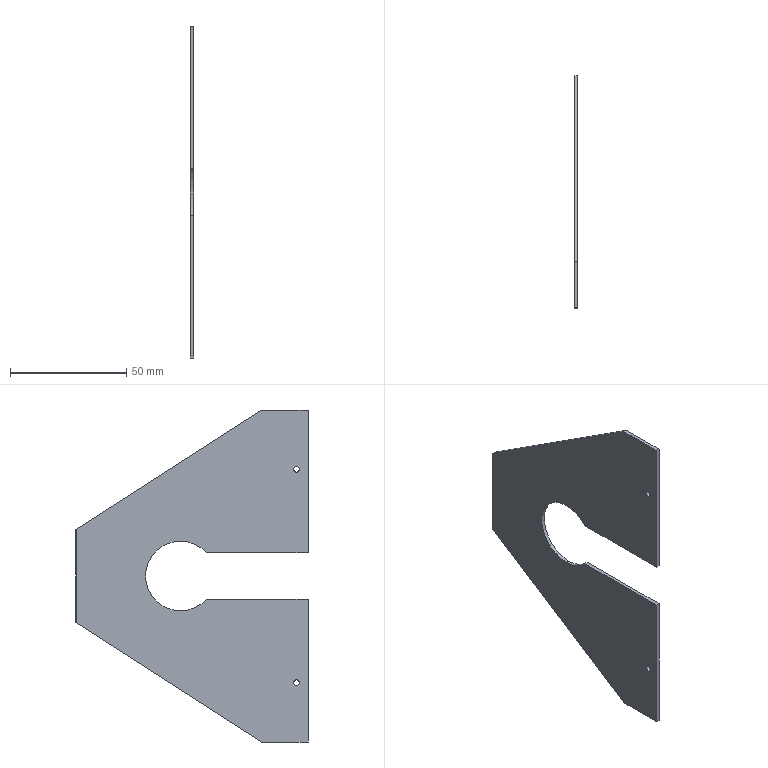Component | SolidWorks | Lampshade-1_Lampshade1-2 | 1 solid | 20 faces | box 1.5 x 100 x 143 mm | volume 12957 mm3 | plane 13 | cylinder 7 | commonest cylinder face diameters 2.5 x4 30 x3
STEP:
#1=CARTESIAN_POINT('',(-6.136,-3.389,1.388));
#2=VERTEX_POINT('',#1);
#3=CARTESIAN_POINT('',(-6.136,-3.389,1.289));
#4=VERTEX_POINT('',#3);
#5=CARTESIAN_POINT('',(-6.136,-3.389,1.339));
#6=DIRECTION('',(1.,-0.,0.));
#7=DIRECTION('',(0.,0.,-1.));
#8=AXIS2_PLACEMENT_3D('',#5,#6,#7);
#9=CIRCLE('',#8,0.04921);
#10=EDGE_CURVE('',#2,#4,#9,.T.);
#11=ORIENTED_EDGE('',*,*,#10,.F.);
#12=CARTESIAN_POINT('',(-6.077,-3.389,1.388));
#13=VERTEX_POINT('',#12);
#14=CARTESIAN_POINT('',(-6.136,-3.389,1.388));
#15=DIRECTION('',(1.,-0.,0.));
#16=VECTOR('',#15,39.37);
#17=LINE('',#14,#16);
#18=EDGE_CURVE('',#2,#13,#17,.T.);
#19=ORIENTED_EDGE('',*,*,#18,.T.);
#20=CARTESIAN_POINT('',(-6.077,-3.389,1.289));
#21=VERTEX_POINT('',#20);
#22=CARTESIAN_POINT('',(-6.077,-3.389,1.339));
#23=DIRECTION('',(1.,-0.,0.));
#24=DIRECTION('',(0.,0.,-1.));
#25=AXIS2_PLACEMENT_3D('',#22,#23,#24);
#26=CIRCLE('',#25,0.04921);
#27=EDGE_CURVE('',#13,#21,#26,.T.);
#28=ORIENTED_EDGE('',*,*,#27,.T.);
#29=CARTESIAN_POINT('',(-6.136,-3.389,1.289));
#30=DIRECTION('',(1.,-0.,0.));
#31=VECTOR('',#30,39.37);
#32=LINE('',#29,#31);
#33=EDGE_CURVE('',#4,#21,#32,.T.);
#34=ORIENTED_EDGE('',*,*,#33,.F.);
#35=EDGE_LOOP('',(#11,#19,#28,#34));
#36=FACE_OUTER_BOUND('',#35,.T.);
#37=CARTESIAN_POINT('',(-6.136,-3.389,1.339));
#38=DIRECTION('',(1.,-0.,0.));
#39=DIRECTION('',(0.,0.,-1.));
#40=AXIS2_PLACEMENT_3D('',#37,#38,#39);
#41=CYLINDRICAL_SURFACE('',#40,0.04921);
#42=ADVANCED_FACE('',(#36),#41,.F.);
#43=CARTESIAN_POINT('',(-6.136,-3.389,5.01));
#44=VERTEX_POINT('',#43);
#45=CARTESIAN_POINT('',(-6.136,-3.389,4.911));
#46=VERTEX_POINT('',#45);
#47=CARTESIAN_POINT('',(-6.136,-3.389,4.961));
#48=DIRECTION('',(1.,-0.,0.));
#49=DIRECTION('',(0.,0.,-1.));
#50=AXIS2_PLACEMENT_3D('',#47,#48,#49);
#51=CIRCLE('',#50,0.04921);
#52=EDGE_CURVE('',#44,#46,#51,.T.);
#53=ORIENTED_EDGE('',*,*,#52,.F.);
#54=CARTESIAN_POINT('',(-6.077,-3.389,5.01));
#55=VERTEX_POINT('',#54);
#56=CARTESIAN_POINT('',(-6.136,-3.389,5.01));
#57=DIRECTION('',(1.,-0.,0.));
#58=VECTOR('',#57,39.37);
#59=LINE('',#56,#58);
#60=EDGE_CURVE('',#44,#55,#59,.T.);
#61=ORIENTED_EDGE('',*,*,#60,.T.);
#62=CARTESIAN_POINT('',(-6.077,-3.389,4.911));
#63=VERTEX_POINT('',#62);
#64=CARTESIAN_POINT('',(-6.077,-3.389,4.961));
#65=DIRECTION('',(1.,-0.,0.));
#66=DIRECTION('',(0.,0.,-1.));
#67=AXIS2_PLACEMENT_3D('',#64,#65,#66);
#68=CIRCLE('',#67,0.04921);
#69=EDGE_CURVE('',#55,#63,#68,.T.);
#70=ORIENTED_EDGE('',*,*,#69,.T.);
#71=CARTESIAN_POINT('',(-6.136,-3.389,4.911));
#72=DIRECTION('',(1.,-0.,0.));
#73=VECTOR('',#72,39.37);
#74=LINE('',#71,#73);
#75=EDGE_CURVE('',#46,#63,#74,.T.);
#76=ORIENTED_EDGE('',*,*,#75,.F.);
#77=EDGE_LOOP('',(#53,#61,#70,#76));
#78=FACE_OUTER_BOUND('',#77,.T.);
#79=CARTESIAN_POINT('',(-6.136,-3.389,4.961));
#80=DIRECTION('',(1.,-0.,0.));
#81=DIRECTION('',(0.,0.,-1.));
#82=AXIS2_PLACEMENT_3D('',#79,#80,#81);
#83=CYLINDRICAL_SURFACE('',#82,0.04921);
#84=ADVANCED_FACE('',(#78),#83,.F.);
#85=CARTESIAN_POINT('',(-6.136,-1.861,3.543));
#86=VERTEX_POINT('',#85);
#87=CARTESIAN_POINT('',(-6.136,-1.421,3.74));
#88=VERTEX_POINT('',#87);
#89=CARTESIAN_POINT('',(-6.136,-1.421,3.15));
#90=DIRECTION('',(-1.,0.,0.));
#91=DIRECTION('',(0.,0.,-1.));
#92=AXIS2_PLACEMENT_3D('',#89,#90,#91);
#93=CIRCLE('',#92,0.5906);
#94=EDGE_CURVE('',#86,#88,#93,.T.);
#95=ORIENTED_EDGE('',*,*,#94,.T.);
#96=CARTESIAN_POINT('',(-6.077,-1.421,3.74));
#97=VERTEX_POINT('',#96);
#98=CARTESIAN_POINT('',(-6.136,-1.421,3.74));
#99=DIRECTION('',(1.,-0.,0.));
#100=VECTOR('',#99,39.37);
#101=LINE('',#98,#100);
#102=EDGE_CURVE('',#88,#97,#101,.T.);
#103=ORIENTED_EDGE('',*,*,#102,.T.);
#104=CARTESIAN_POINT('',(-6.077,-1.861,3.543));
#105=VERTEX_POINT('',#104);
#106=CARTESIAN_POINT('',(-6.077,-1.421,3.15));
#107=DIRECTION('',(-1.,0.,0.));
#108=DIRECTION('',(0.,0.,-1.));
#109=AXIS2_PLACEMENT_3D('',#106,#107,#108);
#110=CIRCLE('',#109,0.5906);
#111=EDGE_CURVE('',#105,#97,#110,.T.);
#112=ORIENTED_EDGE('',*,*,#111,.F.);
#113=CARTESIAN_POINT('',(-6.136,-1.861,3.543));
#114=DIRECTION('',(1.,-0.,0.));
#115=VECTOR('',#114,39.37);
#116=LINE('',#113,#115);
#117=EDGE_CURVE('',#86,#105,#116,.T.);
#118=ORIENTED_EDGE('',*,*,#117,.F.);
#119=EDGE_LOOP('',(#95,#103,#112,#118));
#120=FACE_OUTER_BOUND('',#119,.T.);
#121=CARTESIAN_POINT('',(-6.136,-1.421,3.15));
#122=DIRECTION('',(1.,-0.,0.));
#123=DIRECTION('',(0.,0.,-1.));
#124=AXIS2_PLACEMENT_3D('',#121,#122,#123);
#125=CYLINDRICAL_SURFACE('',#124,0.5906);
#126=ADVANCED_FACE('',(#120),#125,.F.);
#127=ORIENTED_EDGE('',*,*,#102,.F.);
#128=CARTESIAN_POINT('',(-6.136,-1.421,2.559));
#129=VERTEX_POINT('',#128);
#130=CARTESIAN_POINT('',(-6.136,-1.421,3.15));
#131=DIRECTION('',(-1.,0.,0.));
#132=DIRECTION('',(0.,0.,-1.));
#133=AXIS2_PLACEMENT_3D('',#130,#131,#132);
#134=CIRCLE('',#133,0.5906);
#135=EDGE_CURVE('',#88,#129,#134,.T.);
#136=ORIENTED_EDGE('',*,*,#135,.T.);
#137=CARTESIAN_POINT('',(-6.077,-1.421,2.559));
#138=VERTEX_POINT('',#137);
#139=CARTESIAN_POINT('',(-6.136,-1.421,2.559));
#140=DIRECTION('',(1.,-0.,0.));
#141=VECTOR('',#140,39.37);
#142=LINE('',#139,#141);
#143=EDGE_CURVE('',#129,#138,#142,.T.);
#144=ORIENTED_EDGE('',*,*,#143,.T.);
#145=CARTESIAN_POINT('',(-6.077,-1.421,3.15));
#146=DIRECTION('',(-1.,0.,0.));
#147=DIRECTION('',(0.,0.,-1.));
#148=AXIS2_PLACEMENT_3D('',#145,#146,#147);
#149=CIRCLE('',#148,0.5906);
#150=EDGE_CURVE('',#97,#138,#149,.T.);
#151=ORIENTED_EDGE('',*,*,#150,.F.);
#152=EDGE_LOOP('',(#127,#136,#144,#151));
#153=FACE_OUTER_BOUND('',#152,.T.);
#154=CARTESIAN_POINT('',(-6.136,-1.421,3.15));
#155=DIRECTION('',(1.,-0.,0.));
#156=DIRECTION('',(0.,0.,-1.));
#157=AXIS2_PLACEMENT_3D('',#154,#155,#156);
#158=CYLINDRICAL_SURFACE('',#157,0.5906);
#159=ADVANCED_FACE('',(#153),#158,.F.);
#160=CARTESIAN_POINT('',(-6.128,0.3509,2.362));
#161=VERTEX_POINT('',#160);
#162=CARTESIAN_POINT('',(-6.085,0.3509,2.362));
#163=VERTEX_POINT('',#162);
#164=CARTESIAN_POINT('',(-6.136,0.3509,2.362));
#165=DIRECTION('',(1.,-0.,0.));
#166=VECTOR('',#165,39.37);
#167=LINE('',#164,#166);
#168=EDGE_CURVE('',#161,#163,#167,.T.);
#169=ORIENTED_EDGE('',*,*,#168,.T.);
#170=CARTESIAN_POINT('',(-6.077,0.343,2.357));
#171=VERTEX_POINT('',#170);
#172=CARTESIAN_POINT('',(-4.261,-1.473,1.188));
#173=DIRECTION('',(0.6436,-0.6436,-0.4143));
#174=VECTOR('',#173,39.37);
#175=LINE('',#172,#174);
#176=EDGE_CURVE('',#163,#171,#175,.T.);
#177=ORIENTED_EDGE('',*,*,#176,.T.);
#178=CARTESIAN_POINT('',(-6.077,-2.799,0.3346));
#179=VERTEX_POINT('',#178);
#180=CARTESIAN_POINT('',(-6.077,-2.799,0.3346));
#181=DIRECTION('',(0.,0.8408,0.5413));
#182=VECTOR('',#181,39.37);
#183=LINE('',#180,#182);
#184=EDGE_CURVE('',#179,#171,#183,.T.);
#185=ORIENTED_EDGE('',*,*,#184,.F.);
#186=CARTESIAN_POINT('',(-6.136,-2.799,0.3346));
#187=VERTEX_POINT('',#186);
#188=CARTESIAN_POINT('',(-6.136,-2.799,0.3346));
#189=DIRECTION('',(1.,-0.,0.));
#190=VECTOR('',#189,39.37);
#191=LINE('',#188,#190);
#192=EDGE_CURVE('',#187,#179,#191,.T.);
#193=ORIENTED_EDGE('',*,*,#192,.F.);
#194=CARTESIAN_POINT('',(-6.136,0.343,2.357));
#195=VERTEX_POINT('',#194);
#196=CARTESIAN_POINT('',(-6.136,-2.799,0.3346));
#197=DIRECTION('',(0.,0.8408,0.5413));
#198=VECTOR('',#197,39.37);
#199=LINE('',#196,#198);
#200=EDGE_CURVE('',#187,#195,#199,.T.);
#201=ORIENTED_EDGE('',*,*,#200,.T.);
#202=CARTESIAN_POINT('',(-7.977,-1.497,1.172));
#203=DIRECTION('',(0.6436,0.6436,0.4143));
#204=VECTOR('',#203,39.37);
#205=LINE('',#202,#204);
#206=EDGE_CURVE('',#195,#161,#205,.T.);
#207=ORIENTED_EDGE('',*,*,#206,.T.);
#208=EDGE_LOOP('',(#169,#177,#185,#193,#201,#207));
#209=FACE_OUTER_BOUND('',#208,.T.);
#210=CARTESIAN_POINT('',(-6.136,-2.799,0.3346));
#211=DIRECTION('',(0.,0.5413,-0.8408));
#212=DIRECTION('',(0.,0.8408,0.5413));
#213=AXIS2_PLACEMENT_3D('',#210,#211,#212);
#214=PLANE('',#213);
#215=ADVANCED_FACE('',(#209),#214,.T.);
#216=CARTESIAN_POINT('',(-6.077,-3.586,0.3346));
#217=VERTEX_POINT('',#216);
#218=CARTESIAN_POINT('',(-6.077,-3.586,0.3346));
#219=DIRECTION('',(0.,1.,-0.));
#220=VECTOR('',#219,39.37);
#221=LINE('',#218,#220);
#222=EDGE_CURVE('',#217,#179,#221,.T.);
#223=ORIENTED_EDGE('',*,*,#222,.F.);
#224=CARTESIAN_POINT('',(-6.136,-3.586,0.3346));
#225=VERTEX_POINT('',#224);
#226=CARTESIAN_POINT('',(-6.136,-3.586,0.3346));
#227=DIRECTION('',(1.,-0.,0.));
#228=VECTOR('',#227,39.37);
#229=LINE('',#226,#228);
#230=EDGE_CURVE('',#225,#217,#229,.T.);
#231=ORIENTED_EDGE('',*,*,#230,.F.);
#232=CARTESIAN_POINT('',(-6.136,-3.586,0.3346));
#233=DIRECTION('',(0.,1.,-0.));
#234=VECTOR('',#233,39.37);
#235=LINE('',#232,#234);
#236=EDGE_CURVE('',#225,#187,#235,.T.);
#237=ORIENTED_EDGE('',*,*,#236,.T.);
#238=ORIENTED_EDGE('',*,*,#192,.T.);
#239=EDGE_LOOP('',(#223,#231,#237,#238));
#240=FACE_OUTER_BOUND('',#239,.T.);
#241=CARTESIAN_POINT('',(-6.136,-3.586,0.3346));
#242=DIRECTION('',(-0.,-0.,-1.));
#243=DIRECTION('',(-1.,0.,0.));
#244=AXIS2_PLACEMENT_3D('',#241,#242,#243);
#245=PLANE('',#244);
#246=ADVANCED_FACE('',(#240),#245,.T.);
#247=CARTESIAN_POINT('',(-6.077,-3.586,2.756));
#248=VERTEX_POINT('',#247);
#249=CARTESIAN_POINT('',(-6.077,-3.586,2.756));
#250=DIRECTION('',(0.,-0.,-1.));
#251=VECTOR('',#250,39.37);
#252=LINE('',#249,#251);
#253=EDGE_CURVE('',#248,#217,#252,.T.);
#254=ORIENTED_EDGE('',*,*,#253,.F.);
#255=CARTESIAN_POINT('',(-6.136,-3.586,2.756));
#256=VERTEX_POINT('',#255);
#257=CARTESIAN_POINT('',(-6.136,-3.586,2.756));
#258=DIRECTION('',(1.,-0.,0.));
#259=VECTOR('',#258,39.37);
#260=LINE('',#257,#259);
#261=EDGE_CURVE('',#256,#248,#260,.T.);
#262=ORIENTED_EDGE('',*,*,#261,.F.);
#263=CARTESIAN_POINT('',(-6.136,-3.586,2.756));
#264=DIRECTION('',(0.,-0.,-1.));
#265=VECTOR('',#264,39.37);
#266=LINE('',#263,#265);
#267=EDGE_CURVE('',#256,#225,#266,.T.);
#268=ORIENTED_EDGE('',*,*,#267,.T.);
#269=ORIENTED_EDGE('',*,*,#230,.T.);
#270=EDGE_LOOP('',(#254,#262,#268,#269));
#271=FACE_OUTER_BOUND('',#270,.T.);
#272=CARTESIAN_POINT('',(-6.136,-3.586,2.756));
#273=DIRECTION('',(-0.,-1.,0.));
#274=DIRECTION('',(-1.,0.,0.));
#275=AXIS2_PLACEMENT_3D('',#272,#273,#274);
#276=PLANE('',#275);
#277=ADVANCED_FACE('',(#271),#276,.T.);
#278=CARTESIAN_POINT('',(-6.077,-1.861,2.756));
#279=VERTEX_POINT('',#278);
#280=CARTESIAN_POINT('',(-6.077,-1.861,2.756));
#281=DIRECTION('',(-0.,-1.,0.));
#282=VECTOR('',#281,39.37);
#283=LINE('',#280,#282);
#284=EDGE_CURVE('',#279,#248,#283,.T.);
#285=ORIENTED_EDGE('',*,*,#284,.F.);
#286=CARTESIAN_POINT('',(-6.136,-1.861,2.756));
#287=VERTEX_POINT('',#286);
#288=CARTESIAN_POINT('',(-6.136,-1.861,2.756));
#289=DIRECTION('',(1.,-0.,0.));
#290=VECTOR('',#289,39.37);
#291=LINE('',#288,#290);
#292=EDGE_CURVE('',#287,#279,#291,.T.);
#293=ORIENTED_EDGE('',*,*,#292,.F.);
#294=CARTESIAN_POINT('',(-6.136,-1.861,2.756));
#295=DIRECTION('',(-0.,-1.,0.));
#296=VECTOR('',#295,39.37);
#297=LINE('',#294,#296);
#298=EDGE_CURVE('',#287,#256,#297,.T.);
#299=ORIENTED_EDGE('',*,*,#298,.T.);
#300=ORIENTED_EDGE('',*,*,#261,.T.);
#301=EDGE_LOOP('',(#285,#293,#299,#300));
#302=FACE_OUTER_BOUND('',#301,.T.);
#303=CARTESIAN_POINT('',(-6.136,-1.861,2.756));
#304=DIRECTION('',(0.,0.,1.));
#305=DIRECTION('',(1.,-0.,0.));
#306=AXIS2_PLACEMENT_3D('',#303,#304,#305);
#307=PLANE('',#306);
#308=ADVANCED_FACE('',(#302),#307,.T.);
#309=ORIENTED_EDGE('',*,*,#143,.F.);
#310=CARTESIAN_POINT('',(-6.136,-1.421,3.15));
#311=DIRECTION('',(-1.,0.,0.));
#312=DIRECTION('',(0.,0.,-1.));
#313=AXIS2_PLACEMENT_3D('',#310,#311,#312);
#314=CIRCLE('',#313,0.5906);
#315=EDGE_CURVE('',#129,#287,#314,.T.);
#316=ORIENTED_EDGE('',*,*,#315,.T.);
#317=ORIENTED_EDGE('',*,*,#292,.T.);
#318=CARTESIAN_POINT('',(-6.077,-1.421,3.15));
#319=DIRECTION('',(-1.,0.,0.));
#320=DIRECTION('',(0.,0.,-1.));
#321=AXIS2_PLACEMENT_3D('',#318,#319,#320);
#322=CIRCLE('',#321,0.5906);
#323=EDGE_CURVE('',#138,#279,#322,.T.);
#324=ORIENTED_EDGE('',*,*,#323,.F.);
#325=EDGE_LOOP('',(#309,#316,#317,#324));
#326=FACE_OUTER_BOUND('',#325,.T.);
#327=CARTESIAN_POINT('',(-6.136,-1.421,3.15));
#328=DIRECTION('',(1.,-0.,0.));
#329=DIRECTION('',(0.,0.,-1.));
#330=AXIS2_PLACEMENT_3D('',#327,#328,#329);
#331=CYLINDRICAL_SURFACE('',#330,0.5906);
#332=ADVANCED_FACE('',(#326),#331,.F.);
#333=CARTESIAN_POINT('',(-6.077,-3.586,3.543));
#334=VERTEX_POINT('',#333);
#335=CARTESIAN_POINT('',(-6.077,-1.861,3.543));
#336=DIRECTION('',(0.,1.,-0.));
#337=VECTOR('',#336,39.37);
#338=LINE('',#335,#337);
#339=EDGE_CURVE('',#334,#105,#338,.T.);
#340=ORIENTED_EDGE('',*,*,#339,.F.);
#341=CARTESIAN_POINT('',(-6.136,-3.586,3.543));
#342=VERTEX_POINT('',#341);
#343=CARTESIAN_POINT('',(-6.136,-3.586,3.543));
#344=DIRECTION('',(1.,-0.,0.));
#345=VECTOR('',#344,39.37);
#346=LINE('',#343,#345);
#347=EDGE_CURVE('',#342,#334,#346,.T.);
#348=ORIENTED_EDGE('',*,*,#347,.F.);
#349=CARTESIAN_POINT('',(-6.136,-1.861,3.543));
#350=DIRECTION('',(0.,1.,-0.));
#351=VECTOR('',#350,39.37);
#352=LINE('',#349,#351);
#353=EDGE_CURVE('',#342,#86,#352,.T.);
#354=ORIENTED_EDGE('',*,*,#353,.T.);
#355=ORIENTED_EDGE('',*,*,#117,.T.);
#356=EDGE_LOOP('',(#340,#348,#354,#355));
#357=FACE_OUTER_BOUND('',#356,.T.);
#358=CARTESIAN_POINT('',(-6.136,-1.861,3.543));
#359=DIRECTION('',(-0.,-0.,-1.));
#360=DIRECTION('',(-1.,0.,0.));
#361=AXIS2_PLACEMENT_3D('',#358,#359,#360);
#362=PLANE('',#361);
#363=ADVANCED_FACE('',(#357),#362,.T.);
#364=CARTESIAN_POINT('',(-6.077,-3.586,5.965));
#365=VERTEX_POINT('',#364);
#366=CARTESIAN_POINT('',(-6.077,-3.586,5.965));
#367=DIRECTION('',(0.,-0.,-1.));
#368=VECTOR('',#367,39.37);
#369=LINE('',#366,#368);
#370=EDGE_CURVE('',#365,#334,#369,.T.);
#371=ORIENTED_EDGE('',*,*,#370,.F.);
#372=CARTESIAN_POINT('',(-6.136,-3.586,5.965));
#373=VERTEX_POINT('',#372);
#374=CARTESIAN_POINT('',(-6.136,-3.586,5.965));
#375=DIRECTION('',(1.,-0.,0.));
#376=VECTOR('',#375,39.37);
#377=LINE('',#374,#376);
#378=EDGE_CURVE('',#373,#365,#377,.T.);
#379=ORIENTED_EDGE('',*,*,#378,.F.);
#380=CARTESIAN_POINT('',(-6.136,-3.586,5.965));
#381=DIRECTION('',(0.,-0.,-1.));
#382=VECTOR('',#381,39.37);
#383=LINE('',#380,#382);
#384=EDGE_CURVE('',#373,#342,#383,.T.);
#385=ORIENTED_EDGE('',*,*,#384,.T.);
#386=ORIENTED_EDGE('',*,*,#347,.T.);
#387=EDGE_LOOP('',(#371,#379,#385,#386));
#388=FACE_OUTER_BOUND('',#387,.T.);
#389=CARTESIAN_POINT('',(-6.136,-3.586,5.965));
#390=DIRECTION('',(-0.,-1.,0.));
#391=DIRECTION('',(-1.,0.,0.));
#392=AXIS2_PLACEMENT_3D('',#389,#390,#391);
#393=PLANE('',#392);
#394=ADVANCED_FACE('',(#388),#393,.T.);
#395=CARTESIAN_POINT('',(-6.077,-2.799,5.965));
#396=VERTEX_POINT('',#395);
#397=CARTESIAN_POINT('',(-6.077,-2.799,5.965));
#398=DIRECTION('',(-0.,-1.,0.));
#399=VECTOR('',#398,39.37);
#400=LINE('',#397,#399);
#401=EDGE_CURVE('',#396,#365,#400,.T.);
#402=ORIENTED_EDGE('',*,*,#401,.F.);
#403=CARTESIAN_POINT('',(-6.136,-2.799,5.965));
#404=VERTEX_POINT('',#403);
#405=CARTESIAN_POINT('',(-6.136,-2.799,5.965));
#406=DIRECTION('',(1.,-0.,0.));
#407=VECTOR('',#406,39.37);
#408=LINE('',#405,#407);
#409=EDGE_CURVE('',#404,#396,#408,.T.);
#410=ORIENTED_EDGE('',*,*,#409,.F.);
#411=CARTESIAN_POINT('',(-6.136,-2.799,5.965));
#412=DIRECTION('',(-0.,-1.,0.));
#413=VECTOR('',#412,39.37);
#414=LINE('',#411,#413);
#415=EDGE_CURVE('',#404,#373,#414,.T.);
#416=ORIENTED_EDGE('',*,*,#415,.T.);
#417=ORIENTED_EDGE('',*,*,#378,.T.);
#418=EDGE_LOOP('',(#402,#410,#416,#417));
#419=FACE_OUTER_BOUND('',#418,.T.);
#420=CARTESIAN_POINT('',(-6.136,-2.799,5.965));
#421=DIRECTION('',(0.,0.,1.));
#422=DIRECTION('',(1.,-0.,0.));
#423=AXIS2_PLACEMENT_3D('',#420,#421,#422);
#424=PLANE('',#423);
#425=ADVANCED_FACE('',(#419),#424,.T.);
#426=CARTESIAN_POINT('',(-6.077,0.343,3.942));
#427=VERTEX_POINT('',#426);
#428=CARTESIAN_POINT('',(-6.077,0.3509,3.937));
#429=DIRECTION('',(-0.,-0.8408,0.5413));
#430=VECTOR('',#429,39.37);
#431=LINE('',#428,#430);
#432=EDGE_CURVE('',#427,#396,#431,.T.);
#433=ORIENTED_EDGE('',*,*,#432,.F.);
#434=CARTESIAN_POINT('',(-6.085,0.3509,3.937));
#435=VERTEX_POINT('',#434);
#436=CARTESIAN_POINT('',(-6.106,0.3721,3.923));
#437=DIRECTION('',(-0.6436,0.6436,-0.4143));
#438=VECTOR('',#437,39.37);
#439=LINE('',#436,#438);
#440=EDGE_CURVE('',#427,#435,#439,.T.);
#441=ORIENTED_EDGE('',*,*,#440,.T.);
#442=CARTESIAN_POINT('',(-6.128,0.3509,3.937));
#443=VERTEX_POINT('',#442);
#444=CARTESIAN_POINT('',(-6.136,0.3509,3.937));
#445=DIRECTION('',(1.,-0.,0.));
#446=VECTOR('',#445,39.37);
#447=LINE('',#444,#446);
#448=EDGE_CURVE('',#443,#435,#447,.T.);
#449=ORIENTED_EDGE('',*,*,#448,.F.);
#450=CARTESIAN_POINT('',(-6.136,0.343,3.942));
#451=VERTEX_POINT('',#450);
#452=CARTESIAN_POINT('',(-6.132,0.3477,3.939));
#453=DIRECTION('',(-0.6436,-0.6436,0.4143));
#454=VECTOR('',#453,39.37);
#455=LINE('',#452,#454);
#456=EDGE_CURVE('',#443,#451,#455,.T.);
#457=ORIENTED_EDGE('',*,*,#456,.T.);
#458=CARTESIAN_POINT('',(-6.136,0.3509,3.937));
#459=DIRECTION('',(-0.,-0.8408,0.5413));
#460=VECTOR('',#459,39.37);
#461=LINE('',#458,#460);
#462=EDGE_CURVE('',#451,#404,#461,.T.);
#463=ORIENTED_EDGE('',*,*,#462,.T.);
#464=ORIENTED_EDGE('',*,*,#409,.T.);
#465=EDGE_LOOP('',(#433,#441,#449,#457,#463,#464));
#466=FACE_OUTER_BOUND('',#465,.T.);
#467=CARTESIAN_POINT('',(-6.136,0.3509,3.937));
#468=DIRECTION('',(0.,0.5413,0.8408));
#469=DIRECTION('',(-0.,-0.8408,0.5413));
#470=AXIS2_PLACEMENT_3D('',#467,#468,#469);
#471=PLANE('',#470);
#472=ADVANCED_FACE('',(#466),#471,.T.);
#473=ORIENTED_EDGE('',*,*,#448,.T.);
#474=CARTESIAN_POINT('',(-6.085,0.3509,2.362));
#475=DIRECTION('',(0.,0.,-1.));
#476=VECTOR('',#475,39.37);
#477=LINE('',#474,#476);
#478=EDGE_CURVE('',#435,#163,#477,.T.);
#479=ORIENTED_EDGE('',*,*,#478,.T.);
#480=ORIENTED_EDGE('',*,*,#168,.F.);
#481=CARTESIAN_POINT('',(-6.128,0.3509,3.937));
#482=DIRECTION('',(-0.,-0.,1.));
#483=VECTOR('',#482,39.37);
#484=LINE('',#481,#483);
#485=EDGE_CURVE('',#161,#443,#484,.T.);
#486=ORIENTED_EDGE('',*,*,#485,.T.);
#487=EDGE_LOOP('',(#473,#479,#480,#486));
#488=FACE_OUTER_BOUND('',#487,.T.);
#489=CARTESIAN_POINT('',(-6.136,0.3509,2.362));
#490=DIRECTION('',(0.,1.,0.));
#491=DIRECTION('',(-0.,-0.,1.));
#492=AXIS2_PLACEMENT_3D('',#489,#490,#491);
#493=PLANE('',#492);
#494=ADVANCED_FACE('',(#488),#493,.T.);
#495=CARTESIAN_POINT('',(-6.136,-3.389,1.339));
#496=DIRECTION('',(1.,-0.,0.));
#497=DIRECTION('',(0.,0.,-1.));
#498=AXIS2_PLACEMENT_3D('',#495,#496,#497);
#499=CIRCLE('',#498,0.04921);
#500=EDGE_CURVE('',#4,#2,#499,.T.);
#501=ORIENTED_EDGE('',*,*,#500,.T.);
#502=ORIENTED_EDGE('',*,*,#10,.T.);
#503=EDGE_LOOP('',(#501,#502));
#504=FACE_BOUND('',#503,.T.);
#505=CARTESIAN_POINT('',(-6.136,-3.389,4.961));
#506=DIRECTION('',(1.,-0.,0.));
#507=DIRECTION('',(0.,0.,-1.));
#508=AXIS2_PLACEMENT_3D('',#505,#506,#507);
#509=CIRCLE('',#508,0.04921);
#510=EDGE_CURVE('',#46,#44,#509,.T.);
#511=ORIENTED_EDGE('',*,*,#510,.T.);
#512=ORIENTED_EDGE('',*,*,#52,.T.);
#513=EDGE_LOOP('',(#511,#512));
#514=FACE_BOUND('',#513,.T.);
#515=ORIENTED_EDGE('',*,*,#462,.F.);
#516=CARTESIAN_POINT('',(-6.136,0.343,2.362));
#517=DIRECTION('',(0.,0.,-1.));
#518=VECTOR('',#517,39.37);
#519=LINE('',#516,#518);
#520=EDGE_CURVE('',#451,#195,#519,.T.);
#521=ORIENTED_EDGE('',*,*,#520,.T.);
#522=ORIENTED_EDGE('',*,*,#200,.F.);
#523=ORIENTED_EDGE('',*,*,#236,.F.);
#524=ORIENTED_EDGE('',*,*,#267,.F.);
#525=ORIENTED_EDGE('',*,*,#298,.F.);
#526=ORIENTED_EDGE('',*,*,#315,.F.);
#527=ORIENTED_EDGE('',*,*,#135,.F.);
#528=ORIENTED_EDGE('',*,*,#94,.F.);
#529=ORIENTED_EDGE('',*,*,#353,.F.);
#530=ORIENTED_EDGE('',*,*,#384,.F.);
#531=ORIENTED_EDGE('',*,*,#415,.F.);
#532=EDGE_LOOP('',(#515,#521,#522,#523,#524,#525,#526,#527,#528,#529,#530,#531));
#533=FACE_OUTER_BOUND('',#532,.T.);
#534=CARTESIAN_POINT('',(-6.136,-1.421,3.15));
#535=DIRECTION('',(1.,-0.,0.));
#536=DIRECTION('',(0.,-0.,-1.));
#537=AXIS2_PLACEMENT_3D('',#534,#535,#536);
#538=PLANE('',#537);
#539=ADVANCED_FACE('',(#504,#514,#533),#538,.F.);
#540=CARTESIAN_POINT('',(-6.077,-3.389,1.339));
#541=DIRECTION('',(1.,-0.,0.));
#542=DIRECTION('',(0.,0.,-1.));
#543=AXIS2_PLACEMENT_3D('',#540,#541,#542);
#544=CIRCLE('',#543,0.04921);
#545=EDGE_CURVE('',#21,#13,#544,.T.);
#546=ORIENTED_EDGE('',*,*,#545,.F.);
#547=ORIENTED_EDGE('',*,*,#27,.F.);
#548=EDGE_LOOP('',(#546,#547));
#549=FACE_BOUND('',#548,.T.);
#550=CARTESIAN_POINT('',(-6.077,-3.389,4.961));
#551=DIRECTION('',(1.,-0.,0.));
#552=DIRECTION('',(0.,0.,-1.));
#553=AXIS2_PLACEMENT_3D('',#550,#551,#552);
#554=CIRCLE('',#553,0.04921);
#555=EDGE_CURVE('',#63,#55,#554,.T.);
#556=ORIENTED_EDGE('',*,*,#555,.F.);
#557=ORIENTED_EDGE('',*,*,#69,.F.);
#558=EDGE_LOOP('',(#556,#557));
#559=FACE_BOUND('',#558,.T.);
#560=ORIENTED_EDGE('',*,*,#184,.T.);
#561=CARTESIAN_POINT('',(-6.077,0.343,3.15));
#562=DIRECTION('',(-0.,-0.,1.));
#563=VECTOR('',#562,39.37);
#564=LINE('',#561,#563);
#565=EDGE_CURVE('',#171,#427,#564,.T.);
#566=ORIENTED_EDGE('',*,*,#565,.T.);
#567=ORIENTED_EDGE('',*,*,#432,.T.);
#568=ORIENTED_EDGE('',*,*,#401,.T.);
#569=ORIENTED_EDGE('',*,*,#370,.T.);
#570=ORIENTED_EDGE('',*,*,#339,.T.);
#571=ORIENTED_EDGE('',*,*,#111,.T.);
#572=ORIENTED_EDGE('',*,*,#150,.T.);
#573=ORIENTED_EDGE('',*,*,#323,.T.);
#574=ORIENTED_EDGE('',*,*,#284,.T.);
#575=ORIENTED_EDGE('',*,*,#253,.T.);
#576=ORIENTED_EDGE('',*,*,#222,.T.);
#577=EDGE_LOOP('',(#560,#566,#567,#568,#569,#570,#571,#572,#573,#574,#575,#576));
#578=FACE_OUTER_BOUND('',#577,.T.);
#579=CARTESIAN_POINT('',(-6.077,-1.421,3.15));
#580=DIRECTION('',(1.,-0.,0.));
#581=DIRECTION('',(0.,-0.,-1.));
#582=AXIS2_PLACEMENT_3D('',#579,#580,#581);
#583=PLANE('',#582);
#584=ADVANCED_FACE('',(#549,#559,#578),#583,.T.);
#585=ORIENTED_EDGE('',*,*,#60,.F.);
#586=ORIENTED_EDGE('',*,*,#510,.F.);
#587=ORIENTED_EDGE('',*,*,#75,.T.);
#588=ORIENTED_EDGE('',*,*,#555,.T.);
#589=EDGE_LOOP('',(#585,#586,#587,#588));
#590=FACE_OUTER_BOUND('',#589,.T.);
#591=CARTESIAN_POINT('',(-6.136,-3.389,4.961));
#592=DIRECTION('',(1.,-0.,0.));
#593=DIRECTION('',(0.,0.,-1.));
#594=AXIS2_PLACEMENT_3D('',#591,#592,#593);
#595=CYLINDRICAL_SURFACE('',#594,0.04921);
#596=ADVANCED_FACE('',(#590),#595,.F.);
#597=ORIENTED_EDGE('',*,*,#18,.F.);
#598=ORIENTED_EDGE('',*,*,#500,.F.);
#599=ORIENTED_EDGE('',*,*,#33,.T.);
#600=ORIENTED_EDGE('',*,*,#545,.T.);
#601=EDGE_LOOP('',(#597,#598,#599,#600));
#602=FACE_OUTER_BOUND('',#601,.T.);
#603=CARTESIAN_POINT('',(-6.136,-3.389,1.339));
#604=DIRECTION('',(1.,-0.,0.));
#605=DIRECTION('',(0.,0.,-1.));
#606=AXIS2_PLACEMENT_3D('',#603,#604,#605);
#607=CYLINDRICAL_SURFACE('',#606,0.04921);
#608=ADVANCED_FACE('',(#602),#607,.F.);
#609=ORIENTED_EDGE('',*,*,#176,.F.);
#610=ORIENTED_EDGE('',*,*,#478,.F.);
#611=ORIENTED_EDGE('',*,*,#440,.F.);
#612=ORIENTED_EDGE('',*,*,#565,.F.);
#613=EDGE_LOOP('',(#609,#610,#611,#612));
#614=FACE_OUTER_BOUND('',#613,.T.);
#615=CARTESIAN_POINT('',(-6.077,0.343,3.15));
#616=DIRECTION('',(-0.7071,-0.7071,-0.));
#617=DIRECTION('',(-0.,-0.,1.));
#618=AXIS2_PLACEMENT_3D('',#615,#616,#617);
#619=PLANE('',#618);
#620=ADVANCED_FACE('',(#614),#619,.F.);
#621=ORIENTED_EDGE('',*,*,#206,.F.);
#622=ORIENTED_EDGE('',*,*,#520,.F.);
#623=ORIENTED_EDGE('',*,*,#456,.F.);
#624=ORIENTED_EDGE('',*,*,#485,.F.);
#625=EDGE_LOOP('',(#621,#622,#623,#624));
#626=FACE_OUTER_BOUND('',#625,.T.);
#627=CARTESIAN_POINT('',(-6.128,0.3509,2.362));
#628=DIRECTION('',(-0.7071,0.7071,0.));
#629=DIRECTION('',(0.,0.,-1.));
#630=AXIS2_PLACEMENT_3D('',#627,#628,#629);
#631=PLANE('',#630);
#632=ADVANCED_FACE('',(#626),#631,.T.);
#633=CLOSED_SHELL('',(#42,#84,#126,#159,#215,#246,#277,#308,#332,#363,#394,#425,#472,#494,#539,#584,#596,#608,#620,#632));
#634=MANIFOLD_SOLID_BREP('',#633);
#635=CARTESIAN_POINT('',(0.,0.,0.));
#636=DIRECTION('',(0.,0.,1.));
#637=DIRECTION('',(1.,0.,0.));
#638=AXIS2_PLACEMENT_3D('',#635,#636,#637);
#639=(LENGTH_UNIT()NAMED_UNIT(*)SI_UNIT($,.METRE.));
#640=LENGTH_MEASURE_WITH_UNIT(LENGTH_MEASURE(0.0254),#639);
#641=DIMENSIONAL_EXPONENTS(1.,0.,0.,0.,0.,0.,0.);
#642=(CONVERSION_BASED_UNIT('',#640)LENGTH_UNIT()NAMED_UNIT(#641));
#643=UNCERTAINTY_MEASURE_WITH_UNIT(LENGTH_MEASURE(0.00001),#642,'','');
#644=(NAMED_UNIT(*)PLANE_ANGLE_UNIT()SI_UNIT($,.RADIAN.));
#645=(NAMED_UNIT(*)SI_UNIT($,.STERADIAN.)SOLID_ANGLE_UNIT());
#646=(GEOMETRIC_REPRESENTATION_CONTEXT(3)GLOBAL_UNCERTAINTY_ASSIGNED_CONTEXT((#643))GLOBAL_UNIT_ASSIGNED_CONTEXT((#642,#644,#645))REPRESENTATION_CONTEXT('',''));
#647=ADVANCED_BREP_SHAPE_REPRESENTATION('',(#634,#638),#646);
#648=COLOUR_RGB('',0.7922,0.8196,0.9333);
#649=FILL_AREA_STYLE_COLOUR('',#648);
#650=FILL_AREA_STYLE('',(#649));
#651=SURFACE_STYLE_FILL_AREA(#650);
#652=SURFACE_SIDE_STYLE('',(#651));
#653=SURFACE_STYLE_USAGE(.BOTH.,#652);
#654=PRESENTATION_STYLE_ASSIGNMENT((#653));
#655=STYLED_ITEM('',(#654),#634);
#656=PRESENTATION_LAYER_ASSIGNMENT('','',(#655));
#657=(LENGTH_UNIT()NAMED_UNIT(*)SI_UNIT($,.METRE.));
#658=LENGTH_MEASURE_WITH_UNIT(LENGTH_MEASURE(0.0254),#657);
#659=DIMENSIONAL_EXPONENTS(1.,0.,0.,0.,0.,0.,0.);
#660=(CONVERSION_BASED_UNIT('',#658)LENGTH_UNIT()NAMED_UNIT(#659));
#661=UNCERTAINTY_MEASURE_WITH_UNIT(LENGTH_MEASURE(0.00001),#660,'','');
#662=(NAMED_UNIT(*)PLANE_ANGLE_UNIT()SI_UNIT($,.RADIAN.));
#663=(NAMED_UNIT(*)SI_UNIT($,.STERADIAN.)SOLID_ANGLE_UNIT());
#664=(GEOMETRIC_REPRESENTATION_CONTEXT(3)GLOBAL_UNCERTAINTY_ASSIGNED_CONTEXT((#661))GLOBAL_UNIT_ASSIGNED_CONTEXT((#660,#662,#663))REPRESENTATION_CONTEXT('',''));
#665=MECHANICAL_DESIGN_GEOMETRIC_PRESENTATION_REPRESENTATION('',(#655),#664);